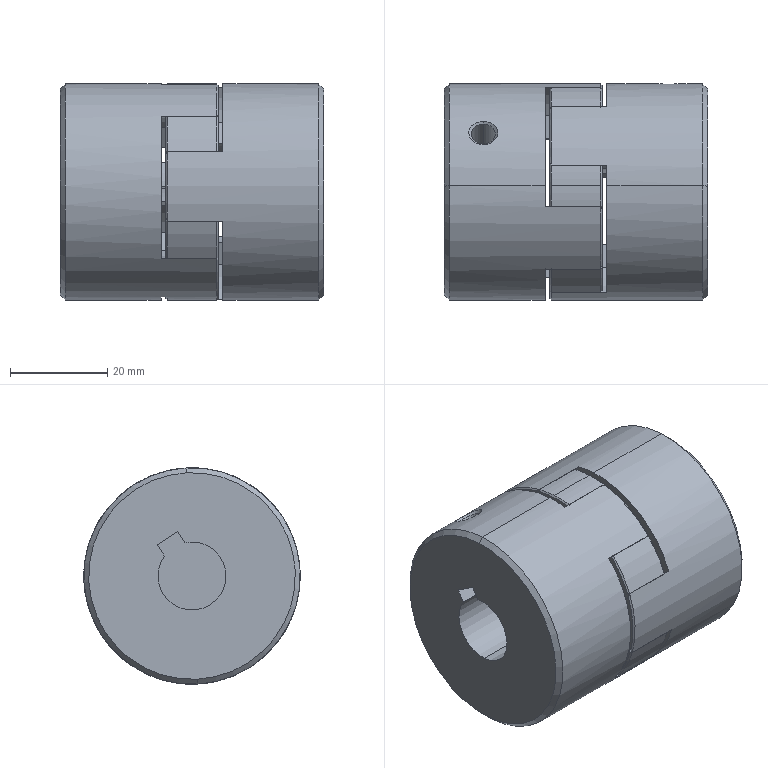Component | SolidWorks | Coupling075-12.7-14-1 | 3 solids | 230 faces | volume 74154 mm3 | cone 87 | plane 75 | cylinder 64 | spline 4 | commonest cylinder face diameters 23.28 x28 22 x12 44.5 x11 12.7 x5 4.917 x4 14 x3 19.26 x1